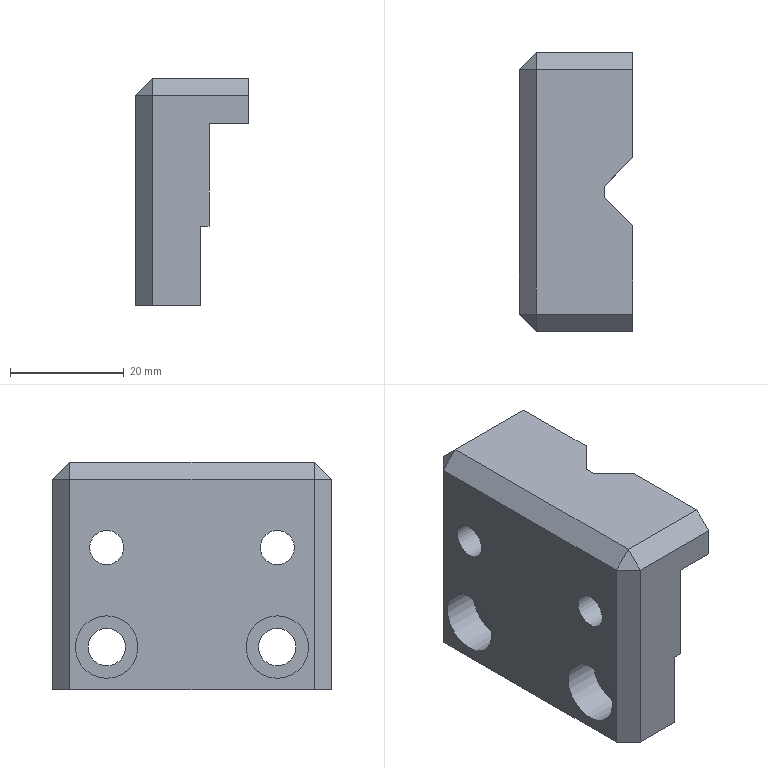Component | NX | FIXED_JAW | 1 solid | 31 faces | volume 23888 mm3 | plane 23 | cylinder 6 | cone 2 | commonest cylinder face diameters 6 x2 6.6 x2 11 x2